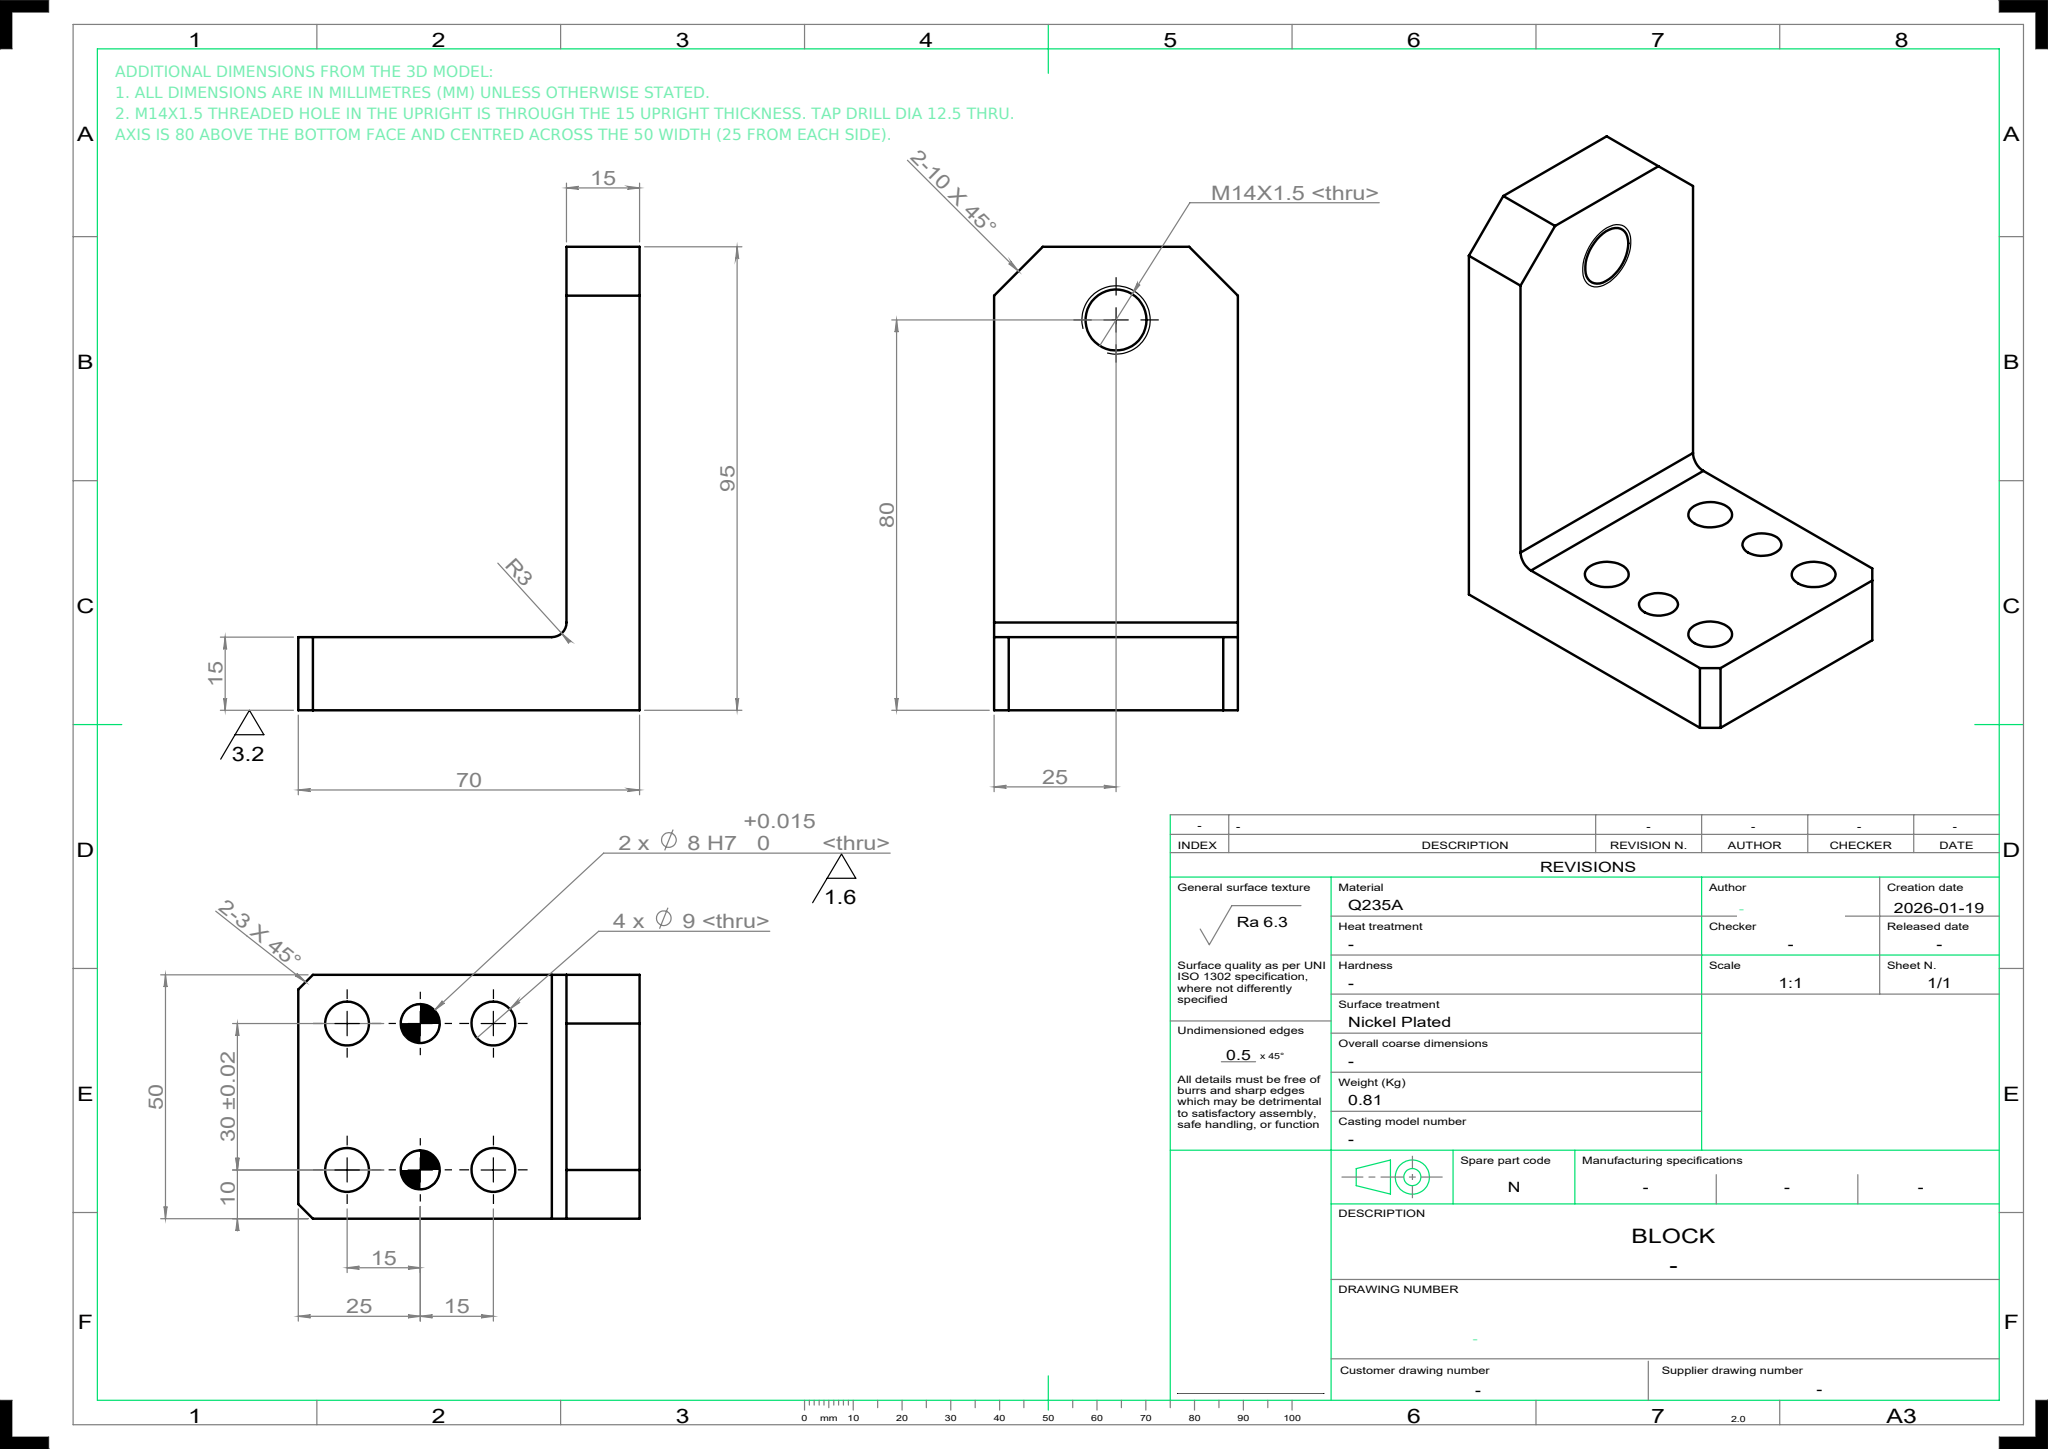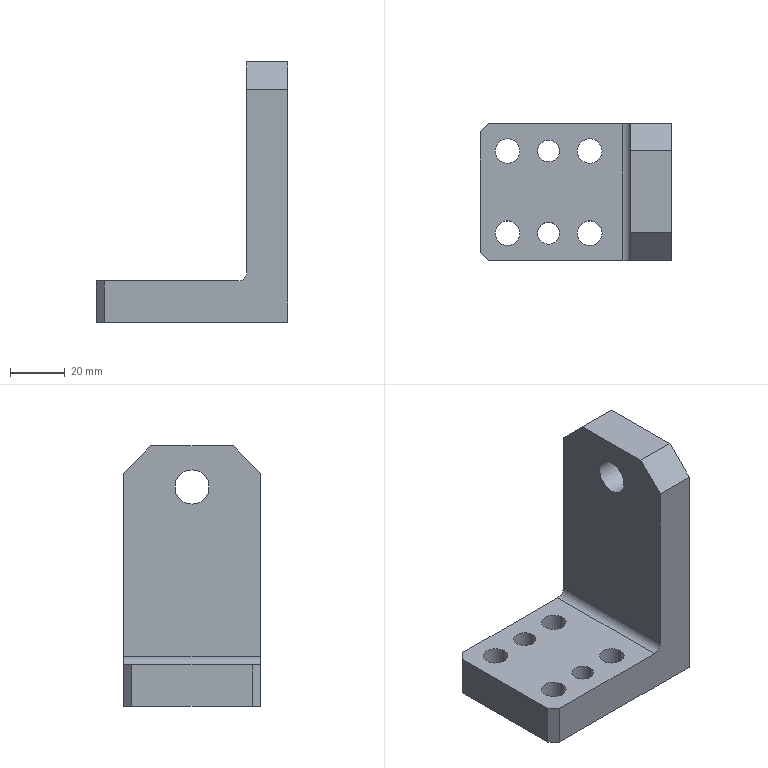Part | NX | mm | 1 solid | 20 faces | box 70 x 50 x 95 mm | volume 103796 mm3 | plane 12 | cylinder 8 | commonest cylinder face diameters 9 x4 8 x2 6 x1 12.5 x1
STEP:
#1=CARTESIAN_POINT('',(0.,0.,0.));
#2=DIRECTION('',(0.,0.,1.));
#3=DIRECTION('',(1.,0.,0.));
#4=AXIS2_PLACEMENT_3D('',#1,#2,#3);
#5=(LENGTH_UNIT()NAMED_UNIT(*)SI_UNIT(.MILLI.,.METRE.));
#6=UNCERTAINTY_MEASURE_WITH_UNIT(LENGTH_MEASURE(0.00002),#5,'','');
#7=(NAMED_UNIT(*)PLANE_ANGLE_UNIT()SI_UNIT($,.RADIAN.));
#8=PLANE_ANGLE_MEASURE_WITH_UNIT(PLANE_ANGLE_MEASURE(0.01745),#7);
#9=DIMENSIONAL_EXPONENTS(0.,0.,0.,0.,0.,0.,0.);
#10=(CONVERSION_BASED_UNIT('',#8)NAMED_UNIT(#9)PLANE_ANGLE_UNIT());
#11=(NAMED_UNIT(*)SI_UNIT($,.STERADIAN.)SOLID_ANGLE_UNIT());
#12=(GEOMETRIC_REPRESENTATION_CONTEXT(3)GLOBAL_UNCERTAINTY_ASSIGNED_CONTEXT((#6))GLOBAL_UNIT_ASSIGNED_CONTEXT((#5,#10,#11))REPRESENTATION_CONTEXT('',''));
#13=SHAPE_REPRESENTATION('',(#4),#12);
#14=CARTESIAN_POINT('',(0.,-0.,86.25));
#15=VERTEX_POINT('',#14);
#16=CARTESIAN_POINT('',(0.,-0.,80.));
#17=DIRECTION('',(-1.,0.,0.));
#18=DIRECTION('',(0.,0.,1.));
#19=AXIS2_PLACEMENT_3D('',#16,#17,#18);
#20=CIRCLE('',#19,6.25);
#21=EDGE_CURVE('',#15,#15,#20,.T.);
#22=ORIENTED_EDGE('',*,*,#21,.T.);
#23=EDGE_LOOP('',(#22));
#24=FACE_BOUND('',#23,.T.);
#25=CARTESIAN_POINT('',(0.,-15.,95.));
#26=VERTEX_POINT('',#25);
#27=CARTESIAN_POINT('',(0.,15.,95.));
#28=VERTEX_POINT('',#27);
#29=CARTESIAN_POINT('',(0.,-25.,95.));
#30=DIRECTION('',(0.,1.,0.));
#31=VECTOR('',#30,1.);
#32=LINE('',#29,#31);
#33=EDGE_CURVE('',#26,#28,#32,.T.);
#34=ORIENTED_EDGE('',*,*,#33,.F.);
#35=CARTESIAN_POINT('',(0.,-25.,85.));
#36=VERTEX_POINT('',#35);
#37=CARTESIAN_POINT('',(0.,-25.,85.));
#38=DIRECTION('',(0.,-0.7071,-0.7071));
#39=VECTOR('',#38,1.);
#40=LINE('',#37,#39);
#41=EDGE_CURVE('',#26,#36,#40,.T.);
#42=ORIENTED_EDGE('',*,*,#41,.T.);
#43=CARTESIAN_POINT('',(0.,-25.,0.));
#44=VERTEX_POINT('',#43);
#45=CARTESIAN_POINT('',(0.,-25.,0.));
#46=DIRECTION('',(0.,0.,1.));
#47=VECTOR('',#46,1.);
#48=LINE('',#45,#47);
#49=EDGE_CURVE('',#44,#36,#48,.T.);
#50=ORIENTED_EDGE('',*,*,#49,.F.);
#51=CARTESIAN_POINT('',(0.,25.,0.));
#52=VERTEX_POINT('',#51);
#53=CARTESIAN_POINT('',(0.,-25.,0.));
#54=DIRECTION('',(0.,1.,0.));
#55=VECTOR('',#54,1.);
#56=LINE('',#53,#55);
#57=EDGE_CURVE('',#44,#52,#56,.T.);
#58=ORIENTED_EDGE('',*,*,#57,.T.);
#59=CARTESIAN_POINT('',(0.,25.,85.));
#60=VERTEX_POINT('',#59);
#61=CARTESIAN_POINT('',(0.,25.,85.));
#62=DIRECTION('',(0.,0.,1.));
#63=VECTOR('',#62,1.);
#64=LINE('',#61,#63);
#65=EDGE_CURVE('',#52,#60,#64,.T.);
#66=ORIENTED_EDGE('',*,*,#65,.T.);
#67=CARTESIAN_POINT('',(0.,15.,95.));
#68=DIRECTION('',(0.,-0.7071,0.7071));
#69=VECTOR('',#68,1.);
#70=LINE('',#67,#69);
#71=EDGE_CURVE('',#60,#28,#70,.T.);
#72=ORIENTED_EDGE('',*,*,#71,.T.);
#73=EDGE_LOOP('',(#34,#42,#50,#58,#66,#72));
#74=FACE_BOUND('',#73,.T.);
#75=CARTESIAN_POINT('',(0.,-25.,85.));
#76=DIRECTION('',(-1.,0.,0.));
#77=DIRECTION('',(0.,0.,1.));
#78=AXIS2_PLACEMENT_3D('',#75,#76,#77);
#79=PLANE('',#78);
#80=ADVANCED_FACE('',(#24,#74),#79,.F.);
#81=CARTESIAN_POINT('',(-15.,-15.,95.));
#82=VERTEX_POINT('',#81);
#83=CARTESIAN_POINT('',(-15.,15.,95.));
#84=VERTEX_POINT('',#83);
#85=CARTESIAN_POINT('',(-15.,-25.,95.));
#86=DIRECTION('',(0.,1.,0.));
#87=VECTOR('',#86,1.);
#88=LINE('',#85,#87);
#89=EDGE_CURVE('',#82,#84,#88,.T.);
#90=ORIENTED_EDGE('',*,*,#89,.F.);
#91=CARTESIAN_POINT('',(0.,-15.,95.));
#92=DIRECTION('',(1.,0.,0.));
#93=VECTOR('',#92,1.);
#94=LINE('',#91,#93);
#95=EDGE_CURVE('',#82,#26,#94,.T.);
#96=ORIENTED_EDGE('',*,*,#95,.T.);
#97=ORIENTED_EDGE('',*,*,#33,.T.);
#98=CARTESIAN_POINT('',(-15.,15.,95.));
#99=DIRECTION('',(-1.,0.,0.));
#100=VECTOR('',#99,1.);
#101=LINE('',#98,#100);
#102=EDGE_CURVE('',#28,#84,#101,.T.);
#103=ORIENTED_EDGE('',*,*,#102,.T.);
#104=EDGE_LOOP('',(#90,#96,#97,#103));
#105=FACE_OUTER_BOUND('',#104,.T.);
#106=CARTESIAN_POINT('',(0.,-25.,95.));
#107=DIRECTION('',(0.,0.,-1.));
#108=DIRECTION('',(-1.,0.,0.));
#109=AXIS2_PLACEMENT_3D('',#106,#107,#108);
#110=PLANE('',#109);
#111=ADVANCED_FACE('',(#105),#110,.F.);
#112=CARTESIAN_POINT('',(-15.,-0.,73.75));
#113=VERTEX_POINT('',#112);
#114=CARTESIAN_POINT('',(-15.,-0.,80.));
#115=DIRECTION('',(1.,0.,0.));
#116=DIRECTION('',(0.,0.,-1.));
#117=AXIS2_PLACEMENT_3D('',#114,#115,#116);
#118=CIRCLE('',#117,6.25);
#119=EDGE_CURVE('',#113,#113,#118,.T.);
#120=ORIENTED_EDGE('',*,*,#119,.T.);
#121=EDGE_LOOP('',(#120));
#122=FACE_BOUND('',#121,.T.);
#123=CARTESIAN_POINT('',(-15.,-25.,85.));
#124=VERTEX_POINT('',#123);
#125=CARTESIAN_POINT('',(-15.,-25.,18.));
#126=VERTEX_POINT('',#125);
#127=CARTESIAN_POINT('',(-15.,-25.,95.));
#128=DIRECTION('',(0.,0.,-1.));
#129=VECTOR('',#128,1.);
#130=LINE('',#127,#129);
#131=EDGE_CURVE('',#124,#126,#130,.T.);
#132=ORIENTED_EDGE('',*,*,#131,.F.);
#133=CARTESIAN_POINT('',(-15.,-25.,85.));
#134=DIRECTION('',(0.,0.7071,0.7071));
#135=VECTOR('',#134,1.);
#136=LINE('',#133,#135);
#137=EDGE_CURVE('',#124,#82,#136,.T.);
#138=ORIENTED_EDGE('',*,*,#137,.T.);
#139=ORIENTED_EDGE('',*,*,#89,.T.);
#140=CARTESIAN_POINT('',(-15.,25.,85.));
#141=VERTEX_POINT('',#140);
#142=CARTESIAN_POINT('',(-15.,15.,95.));
#143=DIRECTION('',(0.,0.7071,-0.7071));
#144=VECTOR('',#143,1.);
#145=LINE('',#142,#144);
#146=EDGE_CURVE('',#84,#141,#145,.T.);
#147=ORIENTED_EDGE('',*,*,#146,.T.);
#148=CARTESIAN_POINT('',(-15.,25.,18.));
#149=VERTEX_POINT('',#148);
#150=CARTESIAN_POINT('',(-15.,25.,85.));
#151=DIRECTION('',(0.,0.,-1.));
#152=VECTOR('',#151,1.);
#153=LINE('',#150,#152);
#154=EDGE_CURVE('',#141,#149,#153,.T.);
#155=ORIENTED_EDGE('',*,*,#154,.T.);
#156=CARTESIAN_POINT('',(-15.,-25.,18.));
#157=DIRECTION('',(0.,1.,0.));
#158=VECTOR('',#157,1.);
#159=LINE('',#156,#158);
#160=EDGE_CURVE('',#126,#149,#159,.T.);
#161=ORIENTED_EDGE('',*,*,#160,.F.);
#162=EDGE_LOOP('',(#132,#138,#139,#147,#155,#161));
#163=FACE_BOUND('',#162,.T.);
#164=CARTESIAN_POINT('',(-15.,-25.,85.));
#165=DIRECTION('',(1.,0.,0.));
#166=DIRECTION('',(0.,0.,-1.));
#167=AXIS2_PLACEMENT_3D('',#164,#165,#166);
#168=PLANE('',#167);
#169=ADVANCED_FACE('',(#122,#163),#168,.F.);
#170=CARTESIAN_POINT('',(-18.,25.,15.));
#171=VERTEX_POINT('',#170);
#172=CARTESIAN_POINT('',(-18.,25.,18.));
#173=DIRECTION('',(0.,1.,0.));
#174=DIRECTION('',(1.,0.,0.));
#175=AXIS2_PLACEMENT_3D('',#172,#173,#174);
#176=CIRCLE('',#175,3.);
#177=EDGE_CURVE('',#149,#171,#176,.T.);
#178=ORIENTED_EDGE('',*,*,#177,.T.);
#179=CARTESIAN_POINT('',(-18.,-25.,15.));
#180=VERTEX_POINT('',#179);
#181=CARTESIAN_POINT('',(-18.,-25.,15.));
#182=DIRECTION('',(0.,1.,0.));
#183=VECTOR('',#182,1.);
#184=LINE('',#181,#183);
#185=EDGE_CURVE('',#180,#171,#184,.T.);
#186=ORIENTED_EDGE('',*,*,#185,.F.);
#187=CARTESIAN_POINT('',(-18.,-25.,18.));
#188=DIRECTION('',(0.,1.,0.));
#189=DIRECTION('',(1.,0.,0.));
#190=AXIS2_PLACEMENT_3D('',#187,#188,#189);
#191=CIRCLE('',#190,3.);
#192=EDGE_CURVE('',#126,#180,#191,.T.);
#193=ORIENTED_EDGE('',*,*,#192,.F.);
#194=ORIENTED_EDGE('',*,*,#160,.T.);
#195=EDGE_LOOP('',(#178,#186,#193,#194));
#196=FACE_OUTER_BOUND('',#195,.T.);
#197=CARTESIAN_POINT('',(-18.,-25.,18.));
#198=DIRECTION('',(0.,1.,0.));
#199=DIRECTION('',(0.,0.,1.));
#200=AXIS2_PLACEMENT_3D('',#197,#198,#199);
#201=CYLINDRICAL_SURFACE('',#200,3.);
#202=ADVANCED_FACE('',(#196),#201,.F.);
#203=CARTESIAN_POINT('',(-34.5,15.,15.));
#204=VERTEX_POINT('',#203);
#205=CARTESIAN_POINT('',(-30.,15.,15.));
#206=DIRECTION('',(0.,0.,-1.));
#207=DIRECTION('',(-1.,0.,0.));
#208=AXIS2_PLACEMENT_3D('',#205,#206,#207);
#209=CIRCLE('',#208,4.5);
#210=EDGE_CURVE('',#204,#204,#209,.T.);
#211=ORIENTED_EDGE('',*,*,#210,.T.);
#212=EDGE_LOOP('',(#211));
#213=FACE_BOUND('',#212,.T.);
#214=CARTESIAN_POINT('',(-34.5,-15.,15.));
#215=VERTEX_POINT('',#214);
#216=CARTESIAN_POINT('',(-30.,-15.,15.));
#217=DIRECTION('',(0.,0.,-1.));
#218=DIRECTION('',(-1.,0.,0.));
#219=AXIS2_PLACEMENT_3D('',#216,#217,#218);
#220=CIRCLE('',#219,4.5);
#221=EDGE_CURVE('',#215,#215,#220,.T.);
#222=ORIENTED_EDGE('',*,*,#221,.T.);
#223=EDGE_LOOP('',(#222));
#224=FACE_BOUND('',#223,.T.);
#225=CARTESIAN_POINT('',(-64.5,15.,15.));
#226=VERTEX_POINT('',#225);
#227=CARTESIAN_POINT('',(-60.,15.,15.));
#228=DIRECTION('',(0.,0.,-1.));
#229=DIRECTION('',(-1.,0.,0.));
#230=AXIS2_PLACEMENT_3D('',#227,#228,#229);
#231=CIRCLE('',#230,4.5);
#232=EDGE_CURVE('',#226,#226,#231,.T.);
#233=ORIENTED_EDGE('',*,*,#232,.T.);
#234=EDGE_LOOP('',(#233));
#235=FACE_BOUND('',#234,.T.);
#236=CARTESIAN_POINT('',(-64.5,-15.,15.));
#237=VERTEX_POINT('',#236);
#238=CARTESIAN_POINT('',(-60.,-15.,15.));
#239=DIRECTION('',(0.,0.,-1.));
#240=DIRECTION('',(-1.,0.,0.));
#241=AXIS2_PLACEMENT_3D('',#238,#239,#240);
#242=CIRCLE('',#241,4.5);
#243=EDGE_CURVE('',#237,#237,#242,.T.);
#244=ORIENTED_EDGE('',*,*,#243,.T.);
#245=EDGE_LOOP('',(#244));
#246=FACE_BOUND('',#245,.T.);
#247=CARTESIAN_POINT('',(-49.,15.,15.));
#248=VERTEX_POINT('',#247);
#249=CARTESIAN_POINT('',(-45.,15.,15.));
#250=DIRECTION('',(0.,0.,-1.));
#251=DIRECTION('',(-1.,0.,0.));
#252=AXIS2_PLACEMENT_3D('',#249,#250,#251);
#253=CIRCLE('',#252,4.);
#254=EDGE_CURVE('',#248,#248,#253,.T.);
#255=ORIENTED_EDGE('',*,*,#254,.T.);
#256=EDGE_LOOP('',(#255));
#257=FACE_BOUND('',#256,.T.);
#258=CARTESIAN_POINT('',(-49.,-15.,15.));
#259=VERTEX_POINT('',#258);
#260=CARTESIAN_POINT('',(-45.,-15.,15.));
#261=DIRECTION('',(0.,0.,-1.));
#262=DIRECTION('',(-1.,0.,0.));
#263=AXIS2_PLACEMENT_3D('',#260,#261,#262);
#264=CIRCLE('',#263,4.);
#265=EDGE_CURVE('',#259,#259,#264,.T.);
#266=ORIENTED_EDGE('',*,*,#265,.T.);
#267=EDGE_LOOP('',(#266));
#268=FACE_BOUND('',#267,.T.);
#269=CARTESIAN_POINT('',(-67.,25.,15.));
#270=VERTEX_POINT('',#269);
#271=CARTESIAN_POINT('',(-18.,25.,15.));
#272=DIRECTION('',(-1.,0.,0.));
#273=VECTOR('',#272,1.);
#274=LINE('',#271,#273);
#275=EDGE_CURVE('',#171,#270,#274,.T.);
#276=ORIENTED_EDGE('',*,*,#275,.T.);
#277=CARTESIAN_POINT('',(-70.,22.,15.));
#278=VERTEX_POINT('',#277);
#279=CARTESIAN_POINT('',(-70.,22.,15.));
#280=DIRECTION('',(-0.7071,-0.7071,0.));
#281=VECTOR('',#280,1.);
#282=LINE('',#279,#281);
#283=EDGE_CURVE('',#270,#278,#282,.T.);
#284=ORIENTED_EDGE('',*,*,#283,.T.);
#285=CARTESIAN_POINT('',(-70.,-22.,15.));
#286=VERTEX_POINT('',#285);
#287=CARTESIAN_POINT('',(-70.,-25.,15.));
#288=DIRECTION('',(0.,1.,0.));
#289=VECTOR('',#288,1.);
#290=LINE('',#287,#289);
#291=EDGE_CURVE('',#286,#278,#290,.T.);
#292=ORIENTED_EDGE('',*,*,#291,.F.);
#293=CARTESIAN_POINT('',(-67.,-25.,15.));
#294=VERTEX_POINT('',#293);
#295=CARTESIAN_POINT('',(-67.,-25.,15.));
#296=DIRECTION('',(0.7071,-0.7071,0.));
#297=VECTOR('',#296,1.);
#298=LINE('',#295,#297);
#299=EDGE_CURVE('',#286,#294,#298,.T.);
#300=ORIENTED_EDGE('',*,*,#299,.T.);
#301=CARTESIAN_POINT('',(-18.,-25.,15.));
#302=DIRECTION('',(-1.,0.,0.));
#303=VECTOR('',#302,1.);
#304=LINE('',#301,#303);
#305=EDGE_CURVE('',#180,#294,#304,.T.);
#306=ORIENTED_EDGE('',*,*,#305,.F.);
#307=ORIENTED_EDGE('',*,*,#185,.T.);
#308=EDGE_LOOP('',(#276,#284,#292,#300,#306,#307));
#309=FACE_BOUND('',#308,.T.);
#310=CARTESIAN_POINT('',(-18.,-25.,15.));
#311=DIRECTION('',(0.,0.,-1.));
#312=DIRECTION('',(-1.,0.,0.));
#313=AXIS2_PLACEMENT_3D('',#310,#311,#312);
#314=PLANE('',#313);
#315=ADVANCED_FACE('',(#213,#224,#235,#246,#257,#268,#309),#314,.F.);
#316=ORIENTED_EDGE('',*,*,#291,.T.);
#317=CARTESIAN_POINT('',(-70.,22.,0.));
#318=VERTEX_POINT('',#317);
#319=CARTESIAN_POINT('',(-70.,22.,0.));
#320=DIRECTION('',(0.,0.,-1.));
#321=VECTOR('',#320,1.);
#322=LINE('',#319,#321);
#323=EDGE_CURVE('',#278,#318,#322,.T.);
#324=ORIENTED_EDGE('',*,*,#323,.T.);
#325=CARTESIAN_POINT('',(-70.,-22.,0.));
#326=VERTEX_POINT('',#325);
#327=CARTESIAN_POINT('',(-70.,-25.,0.));
#328=DIRECTION('',(0.,1.,0.));
#329=VECTOR('',#328,1.);
#330=LINE('',#327,#329);
#331=EDGE_CURVE('',#326,#318,#330,.T.);
#332=ORIENTED_EDGE('',*,*,#331,.F.);
#333=CARTESIAN_POINT('',(-70.,-22.,15.));
#334=DIRECTION('',(0.,0.,1.));
#335=VECTOR('',#334,1.);
#336=LINE('',#333,#335);
#337=EDGE_CURVE('',#326,#286,#336,.T.);
#338=ORIENTED_EDGE('',*,*,#337,.T.);
#339=EDGE_LOOP('',(#316,#324,#332,#338));
#340=FACE_OUTER_BOUND('',#339,.T.);
#341=CARTESIAN_POINT('',(-70.,-25.,15.));
#342=DIRECTION('',(1.,0.,0.));
#343=DIRECTION('',(0.,0.,-1.));
#344=AXIS2_PLACEMENT_3D('',#341,#342,#343);
#345=PLANE('',#344);
#346=ADVANCED_FACE('',(#340),#345,.F.);
#347=CARTESIAN_POINT('',(-25.5,15.,0.));
#348=VERTEX_POINT('',#347);
#349=CARTESIAN_POINT('',(-30.,15.,0.));
#350=DIRECTION('',(0.,0.,1.));
#351=DIRECTION('',(1.,0.,0.));
#352=AXIS2_PLACEMENT_3D('',#349,#350,#351);
#353=CIRCLE('',#352,4.5);
#354=EDGE_CURVE('',#348,#348,#353,.T.);
#355=ORIENTED_EDGE('',*,*,#354,.T.);
#356=EDGE_LOOP('',(#355));
#357=FACE_BOUND('',#356,.T.);
#358=CARTESIAN_POINT('',(-25.5,-15.,0.));
#359=VERTEX_POINT('',#358);
#360=CARTESIAN_POINT('',(-30.,-15.,0.));
#361=DIRECTION('',(0.,0.,1.));
#362=DIRECTION('',(1.,0.,0.));
#363=AXIS2_PLACEMENT_3D('',#360,#361,#362);
#364=CIRCLE('',#363,4.5);
#365=EDGE_CURVE('',#359,#359,#364,.T.);
#366=ORIENTED_EDGE('',*,*,#365,.T.);
#367=EDGE_LOOP('',(#366));
#368=FACE_BOUND('',#367,.T.);
#369=CARTESIAN_POINT('',(-55.5,15.,0.));
#370=VERTEX_POINT('',#369);
#371=CARTESIAN_POINT('',(-60.,15.,0.));
#372=DIRECTION('',(0.,0.,1.));
#373=DIRECTION('',(1.,0.,0.));
#374=AXIS2_PLACEMENT_3D('',#371,#372,#373);
#375=CIRCLE('',#374,4.5);
#376=EDGE_CURVE('',#370,#370,#375,.T.);
#377=ORIENTED_EDGE('',*,*,#376,.T.);
#378=EDGE_LOOP('',(#377));
#379=FACE_BOUND('',#378,.T.);
#380=CARTESIAN_POINT('',(-55.5,-15.,0.));
#381=VERTEX_POINT('',#380);
#382=CARTESIAN_POINT('',(-60.,-15.,0.));
#383=DIRECTION('',(0.,0.,1.));
#384=DIRECTION('',(1.,0.,0.));
#385=AXIS2_PLACEMENT_3D('',#382,#383,#384);
#386=CIRCLE('',#385,4.5);
#387=EDGE_CURVE('',#381,#381,#386,.T.);
#388=ORIENTED_EDGE('',*,*,#387,.T.);
#389=EDGE_LOOP('',(#388));
#390=FACE_BOUND('',#389,.T.);
#391=CARTESIAN_POINT('',(-41.,15.,0.));
#392=VERTEX_POINT('',#391);
#393=CARTESIAN_POINT('',(-45.,15.,0.));
#394=DIRECTION('',(0.,0.,1.));
#395=DIRECTION('',(1.,0.,0.));
#396=AXIS2_PLACEMENT_3D('',#393,#394,#395);
#397=CIRCLE('',#396,4.);
#398=EDGE_CURVE('',#392,#392,#397,.T.);
#399=ORIENTED_EDGE('',*,*,#398,.T.);
#400=EDGE_LOOP('',(#399));
#401=FACE_BOUND('',#400,.T.);
#402=CARTESIAN_POINT('',(-41.,-15.,0.));
#403=VERTEX_POINT('',#402);
#404=CARTESIAN_POINT('',(-45.,-15.,0.));
#405=DIRECTION('',(0.,0.,1.));
#406=DIRECTION('',(1.,0.,0.));
#407=AXIS2_PLACEMENT_3D('',#404,#405,#406);
#408=CIRCLE('',#407,4.);
#409=EDGE_CURVE('',#403,#403,#408,.T.);
#410=ORIENTED_EDGE('',*,*,#409,.T.);
#411=EDGE_LOOP('',(#410));
#412=FACE_BOUND('',#411,.T.);
#413=ORIENTED_EDGE('',*,*,#331,.T.);
#414=CARTESIAN_POINT('',(-67.,25.,0.));
#415=VERTEX_POINT('',#414);
#416=CARTESIAN_POINT('',(-70.,22.,0.));
#417=DIRECTION('',(0.7071,0.7071,0.));
#418=VECTOR('',#417,1.);
#419=LINE('',#416,#418);
#420=EDGE_CURVE('',#318,#415,#419,.T.);
#421=ORIENTED_EDGE('',*,*,#420,.T.);
#422=CARTESIAN_POINT('',(-67.,25.,0.));
#423=DIRECTION('',(1.,0.,0.));
#424=VECTOR('',#423,1.);
#425=LINE('',#422,#424);
#426=EDGE_CURVE('',#415,#52,#425,.T.);
#427=ORIENTED_EDGE('',*,*,#426,.T.);
#428=ORIENTED_EDGE('',*,*,#57,.F.);
#429=CARTESIAN_POINT('',(-67.,-25.,0.));
#430=VERTEX_POINT('',#429);
#431=CARTESIAN_POINT('',(-70.,-25.,0.));
#432=DIRECTION('',(1.,0.,0.));
#433=VECTOR('',#432,1.);
#434=LINE('',#431,#433);
#435=EDGE_CURVE('',#430,#44,#434,.T.);
#436=ORIENTED_EDGE('',*,*,#435,.F.);
#437=CARTESIAN_POINT('',(-67.,-25.,0.));
#438=DIRECTION('',(-0.7071,0.7071,0.));
#439=VECTOR('',#438,1.);
#440=LINE('',#437,#439);
#441=EDGE_CURVE('',#430,#326,#440,.T.);
#442=ORIENTED_EDGE('',*,*,#441,.T.);
#443=EDGE_LOOP('',(#413,#421,#427,#428,#436,#442));
#444=FACE_BOUND('',#443,.T.);
#445=CARTESIAN_POINT('',(-67.,-25.,0.));
#446=DIRECTION('',(0.,0.,1.));
#447=DIRECTION('',(1.,0.,0.));
#448=AXIS2_PLACEMENT_3D('',#445,#446,#447);
#449=PLANE('',#448);
#450=ADVANCED_FACE('',(#357,#368,#379,#390,#401,#412,#444),#449,.F.);
#451=ORIENTED_EDGE('',*,*,#49,.T.);
#452=CARTESIAN_POINT('',(-18.,-25.,85.));
#453=DIRECTION('',(-1.,0.,0.));
#454=VECTOR('',#453,1.);
#455=LINE('',#452,#454);
#456=EDGE_CURVE('',#36,#124,#455,.T.);
#457=ORIENTED_EDGE('',*,*,#456,.T.);
#458=ORIENTED_EDGE('',*,*,#131,.T.);
#459=ORIENTED_EDGE('',*,*,#192,.T.);
#460=ORIENTED_EDGE('',*,*,#305,.T.);
#461=CARTESIAN_POINT('',(-67.,-25.,18.));
#462=DIRECTION('',(0.,0.,-1.));
#463=VECTOR('',#462,1.);
#464=LINE('',#461,#463);
#465=EDGE_CURVE('',#294,#430,#464,.T.);
#466=ORIENTED_EDGE('',*,*,#465,.T.);
#467=ORIENTED_EDGE('',*,*,#435,.T.);
#468=EDGE_LOOP('',(#451,#457,#458,#459,#460,#466,#467));
#469=FACE_OUTER_BOUND('',#468,.T.);
#470=CARTESIAN_POINT('',(-18.,-25.,18.));
#471=DIRECTION('',(0.,1.,0.));
#472=DIRECTION('',(0.,0.,1.));
#473=AXIS2_PLACEMENT_3D('',#470,#471,#472);
#474=PLANE('',#473);
#475=ADVANCED_FACE('',(#469),#474,.F.);
#476=ORIENTED_EDGE('',*,*,#154,.F.);
#477=CARTESIAN_POINT('',(0.,25.,85.));
#478=DIRECTION('',(1.,0.,0.));
#479=VECTOR('',#478,1.);
#480=LINE('',#477,#479);
#481=EDGE_CURVE('',#141,#60,#480,.T.);
#482=ORIENTED_EDGE('',*,*,#481,.T.);
#483=ORIENTED_EDGE('',*,*,#65,.F.);
#484=ORIENTED_EDGE('',*,*,#426,.F.);
#485=CARTESIAN_POINT('',(-67.,25.,15.));
#486=DIRECTION('',(0.,0.,1.));
#487=VECTOR('',#486,1.);
#488=LINE('',#485,#487);
#489=EDGE_CURVE('',#415,#270,#488,.T.);
#490=ORIENTED_EDGE('',*,*,#489,.T.);
#491=ORIENTED_EDGE('',*,*,#275,.F.);
#492=ORIENTED_EDGE('',*,*,#177,.F.);
#493=EDGE_LOOP('',(#476,#482,#483,#484,#490,#491,#492));
#494=FACE_OUTER_BOUND('',#493,.T.);
#495=CARTESIAN_POINT('',(-18.,25.,18.));
#496=DIRECTION('',(0.,1.,0.));
#497=DIRECTION('',(0.,0.,1.));
#498=AXIS2_PLACEMENT_3D('',#495,#496,#497);
#499=PLANE('',#498);
#500=ADVANCED_FACE('',(#494),#499,.T.);
#501=ORIENTED_EDGE('',*,*,#41,.F.);
#502=ORIENTED_EDGE('',*,*,#95,.F.);
#503=ORIENTED_EDGE('',*,*,#137,.F.);
#504=ORIENTED_EDGE('',*,*,#456,.F.);
#505=EDGE_LOOP('',(#501,#502,#503,#504));
#506=FACE_OUTER_BOUND('',#505,.T.);
#507=CARTESIAN_POINT('',(-18.,-25.,85.));
#508=DIRECTION('',(0.,0.7071,-0.7071));
#509=DIRECTION('',(-1.,0.,0.));
#510=AXIS2_PLACEMENT_3D('',#507,#508,#509);
#511=PLANE('',#510);
#512=ADVANCED_FACE('',(#506),#511,.F.);
#513=ORIENTED_EDGE('',*,*,#71,.F.);
#514=ORIENTED_EDGE('',*,*,#481,.F.);
#515=ORIENTED_EDGE('',*,*,#146,.F.);
#516=ORIENTED_EDGE('',*,*,#102,.F.);
#517=EDGE_LOOP('',(#513,#514,#515,#516));
#518=FACE_OUTER_BOUND('',#517,.T.);
#519=CARTESIAN_POINT('',(0.,15.,95.));
#520=DIRECTION('',(0.,0.7071,0.7071));
#521=DIRECTION('',(1.,0.,0.));
#522=AXIS2_PLACEMENT_3D('',#519,#520,#521);
#523=PLANE('',#522);
#524=ADVANCED_FACE('',(#518),#523,.T.);
#525=ORIENTED_EDGE('',*,*,#283,.F.);
#526=ORIENTED_EDGE('',*,*,#489,.F.);
#527=ORIENTED_EDGE('',*,*,#420,.F.);
#528=ORIENTED_EDGE('',*,*,#323,.F.);
#529=EDGE_LOOP('',(#525,#526,#527,#528));
#530=FACE_OUTER_BOUND('',#529,.T.);
#531=CARTESIAN_POINT('',(-70.,22.,15.));
#532=DIRECTION('',(-0.7071,0.7071,0.));
#533=DIRECTION('',(0.,0.,1.));
#534=AXIS2_PLACEMENT_3D('',#531,#532,#533);
#535=PLANE('',#534);
#536=ADVANCED_FACE('',(#530),#535,.T.);
#537=ORIENTED_EDGE('',*,*,#299,.F.);
#538=ORIENTED_EDGE('',*,*,#337,.F.);
#539=ORIENTED_EDGE('',*,*,#441,.F.);
#540=ORIENTED_EDGE('',*,*,#465,.F.);
#541=EDGE_LOOP('',(#537,#538,#539,#540));
#542=FACE_OUTER_BOUND('',#541,.T.);
#543=CARTESIAN_POINT('',(-67.,-25.,18.));
#544=DIRECTION('',(0.7071,0.7071,0.));
#545=DIRECTION('',(0.,0.,-1.));
#546=AXIS2_PLACEMENT_3D('',#543,#544,#545);
#547=PLANE('',#546);
#548=ADVANCED_FACE('',(#542),#547,.F.);
#549=ORIENTED_EDGE('',*,*,#409,.F.);
#550=EDGE_LOOP('',(#549));
#551=FACE_BOUND('',#550,.T.);
#552=ORIENTED_EDGE('',*,*,#265,.F.);
#553=EDGE_LOOP('',(#552));
#554=FACE_BOUND('',#553,.T.);
#555=CARTESIAN_POINT('',(-45.,-15.,0.));
#556=DIRECTION('',(0.,0.,1.));
#557=DIRECTION('',(1.,0.,0.));
#558=AXIS2_PLACEMENT_3D('',#555,#556,#557);
#559=CYLINDRICAL_SURFACE('',#558,4.);
#560=ADVANCED_FACE('',(#551,#554),#559,.F.);
#561=ORIENTED_EDGE('',*,*,#398,.F.);
#562=EDGE_LOOP('',(#561));
#563=FACE_BOUND('',#562,.T.);
#564=ORIENTED_EDGE('',*,*,#254,.F.);
#565=EDGE_LOOP('',(#564));
#566=FACE_BOUND('',#565,.T.);
#567=CARTESIAN_POINT('',(-45.,15.,0.));
#568=DIRECTION('',(0.,0.,1.));
#569=DIRECTION('',(1.,0.,0.));
#570=AXIS2_PLACEMENT_3D('',#567,#568,#569);
#571=CYLINDRICAL_SURFACE('',#570,4.);
#572=ADVANCED_FACE('',(#563,#566),#571,.F.);
#573=ORIENTED_EDGE('',*,*,#387,.F.);
#574=EDGE_LOOP('',(#573));
#575=FACE_BOUND('',#574,.T.);
#576=ORIENTED_EDGE('',*,*,#243,.F.);
#577=EDGE_LOOP('',(#576));
#578=FACE_BOUND('',#577,.T.);
#579=CARTESIAN_POINT('',(-60.,-15.,0.));
#580=DIRECTION('',(0.,0.,1.));
#581=DIRECTION('',(1.,0.,0.));
#582=AXIS2_PLACEMENT_3D('',#579,#580,#581);
#583=CYLINDRICAL_SURFACE('',#582,4.5);
#584=ADVANCED_FACE('',(#575,#578),#583,.F.);
#585=ORIENTED_EDGE('',*,*,#376,.F.);
#586=EDGE_LOOP('',(#585));
#587=FACE_BOUND('',#586,.T.);
#588=ORIENTED_EDGE('',*,*,#232,.F.);
#589=EDGE_LOOP('',(#588));
#590=FACE_BOUND('',#589,.T.);
#591=CARTESIAN_POINT('',(-60.,15.,0.));
#592=DIRECTION('',(0.,0.,1.));
#593=DIRECTION('',(1.,0.,0.));
#594=AXIS2_PLACEMENT_3D('',#591,#592,#593);
#595=CYLINDRICAL_SURFACE('',#594,4.5);
#596=ADVANCED_FACE('',(#587,#590),#595,.F.);
#597=ORIENTED_EDGE('',*,*,#365,.F.);
#598=EDGE_LOOP('',(#597));
#599=FACE_BOUND('',#598,.T.);
#600=ORIENTED_EDGE('',*,*,#221,.F.);
#601=EDGE_LOOP('',(#600));
#602=FACE_BOUND('',#601,.T.);
#603=CARTESIAN_POINT('',(-30.,-15.,0.));
#604=DIRECTION('',(0.,0.,1.));
#605=DIRECTION('',(1.,0.,0.));
#606=AXIS2_PLACEMENT_3D('',#603,#604,#605);
#607=CYLINDRICAL_SURFACE('',#606,4.5);
#608=ADVANCED_FACE('',(#599,#602),#607,.F.);
#609=ORIENTED_EDGE('',*,*,#354,.F.);
#610=EDGE_LOOP('',(#609));
#611=FACE_BOUND('',#610,.T.);
#612=ORIENTED_EDGE('',*,*,#210,.F.);
#613=EDGE_LOOP('',(#612));
#614=FACE_BOUND('',#613,.T.);
#615=CARTESIAN_POINT('',(-30.,15.,0.));
#616=DIRECTION('',(0.,0.,1.));
#617=DIRECTION('',(1.,0.,0.));
#618=AXIS2_PLACEMENT_3D('',#615,#616,#617);
#619=CYLINDRICAL_SURFACE('',#618,4.5);
#620=ADVANCED_FACE('',(#611,#614),#619,.F.);
#621=ORIENTED_EDGE('',*,*,#21,.F.);
#622=EDGE_LOOP('',(#621));
#623=FACE_BOUND('',#622,.T.);
#624=ORIENTED_EDGE('',*,*,#119,.F.);
#625=EDGE_LOOP('',(#624));
#626=FACE_BOUND('',#625,.T.);
#627=CARTESIAN_POINT('',(0.,-0.,80.));
#628=DIRECTION('',(-1.,0.,0.));
#629=DIRECTION('',(0.,0.,1.));
#630=AXIS2_PLACEMENT_3D('',#627,#628,#629);
#631=CYLINDRICAL_SURFACE('',#630,6.25);
#632=ADVANCED_FACE('',(#623,#626),#631,.F.);
#633=CLOSED_SHELL('',(#80,#111,#169,#202,#315,#346,#450,#475,#500,#512,#524,#536,#548,#560,#572,#584,#596,#608,#620,#632));
#634=MANIFOLD_SOLID_BREP('',#633);
#635=ADVANCED_BREP_SHAPE_REPRESENTATION('',(#634),#12);
#636=SHAPE_REPRESENTATION_RELATIONSHIP('','',#13,#635);
#637=PRESENTATION_LAYER_ASSIGNMENT('','',(#634));
#638=COLOUR_RGB('',0.4,0.8,1.);
#639=FILL_AREA_STYLE_COLOUR('',#638);
#640=FILL_AREA_STYLE('',(#639));
#641=SURFACE_STYLE_FILL_AREA(#640);
#642=SURFACE_SIDE_STYLE('',(#641));
#643=SURFACE_STYLE_USAGE(.BOTH.,#642);
#644=PRESENTATION_STYLE_ASSIGNMENT((#643));
#645=STYLED_ITEM('',(#644),#634);
#646=MECHANICAL_DESIGN_GEOMETRIC_PRESENTATION_REPRESENTATION('',(#645),#12);